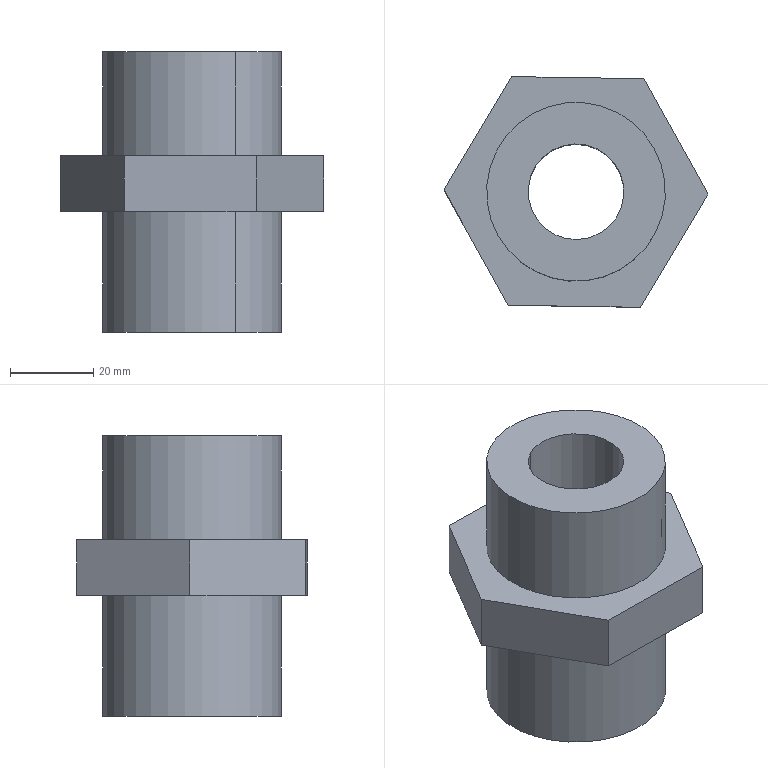Component | SolidWorks | YC1-250-04BalancerAssembly#16673-1_Rc11-4StraightInternalConnection-1 | 1 solid | 16 faces | box 63.5 x 55.49 x 67.5 mm | volume 85682 mm3 | plane 10 | cylinder 6 | commonest cylinder face diameters 43 x4 23 x2 | material Plain Carbon Steel
STEP:
#1=COLOUR_RGB('',0.7922,0.8196,0.9333);
#2=FILL_AREA_STYLE_COLOUR('',#1);
#3=FILL_AREA_STYLE('',(#2));
#4=SURFACE_STYLE_FILL_AREA(#3);
#5=SURFACE_SIDE_STYLE('',(#4));
#6=SURFACE_STYLE_USAGE(.BOTH.,#5);
#7=PRESENTATION_STYLE_ASSIGNMENT((#6));
#8=CARTESIAN_POINT('',(-18.331,156.793,-8.484));
#9=VERTEX_POINT('',#8);
#10=CARTESIAN_POINT('',(-17.89,156.002,-8.484));
#11=VERTEX_POINT('',#10);
#12=CARTESIAN_POINT('',(-18.11,156.398,-8.484));
#13=DIRECTION('',(-0.,-0.,-1.));
#14=DIRECTION('',(-0.8737,-0.4865,0.));
#15=AXIS2_PLACEMENT_3D('',#12,#13,#14);
#16=CIRCLE('',#15,0.4528);
#17=EDGE_CURVE('',#9,#11,#16,.T.);
#18=ORIENTED_EDGE('',*,*,#17,.T.);
#19=CARTESIAN_POINT('',(-17.89,156.002,-5.827));
#20=VERTEX_POINT('',#19);
#21=CARTESIAN_POINT('',(-17.89,156.002,-8.583));
#22=DIRECTION('',(0.,0.,1.));
#23=VECTOR('',#22,39.37);
#24=LINE('',#21,#23);
#25=EDGE_CURVE('',#11,#20,#24,.T.);
#26=ORIENTED_EDGE('',*,*,#25,.T.);
#27=CARTESIAN_POINT('',(-18.331,156.793,-5.827));
#28=VERTEX_POINT('',#27);
#29=CARTESIAN_POINT('',(-18.11,156.398,-5.827));
#30=DIRECTION('',(-0.,-0.,-1.));
#31=DIRECTION('',(-0.4865,0.8737,0.));
#32=AXIS2_PLACEMENT_3D('',#29,#30,#31);
#33=CIRCLE('',#32,0.4528);
#34=EDGE_CURVE('',#28,#20,#33,.T.);
#35=ORIENTED_EDGE('',*,*,#34,.F.);
#36=CARTESIAN_POINT('',(-18.331,156.793,-8.583));
#37=DIRECTION('',(0.,0.,1.));
#38=VECTOR('',#37,39.37);
#39=LINE('',#36,#38);
#40=EDGE_CURVE('',#9,#28,#39,.T.);
#41=ORIENTED_EDGE('',*,*,#40,.F.);
#42=EDGE_LOOP('',(#18,#26,#35,#41));
#43=FACE_OUTER_BOUND('',#42,.T.);
#44=CARTESIAN_POINT('',(-18.11,156.398,-8.583));
#45=DIRECTION('',(0.,0.,1.));
#46=DIRECTION('',(-0.4865,0.8737,0.));
#47=AXIS2_PLACEMENT_3D('',#44,#45,#46);
#48=CYLINDRICAL_SURFACE('',#47,0.4528);
#49=ADVANCED_FACE('',(#43),#48,.F.);
#50=CARTESIAN_POINT('',(-17.698,155.658,-8.484));
#51=VERTEX_POINT('',#50);
#52=CARTESIAN_POINT('',(-18.522,157.137,-8.484));
#53=VERTEX_POINT('',#52);
#54=CARTESIAN_POINT('',(-18.11,156.398,-8.484));
#55=DIRECTION('',(-0.,-0.,-1.));
#56=DIRECTION('',(-0.8737,-0.4865,0.));
#57=AXIS2_PLACEMENT_3D('',#54,#55,#56);
#58=CIRCLE('',#57,0.8465);
#59=EDGE_CURVE('',#51,#53,#58,.T.);
#60=ORIENTED_EDGE('',*,*,#59,.F.);
#61=CARTESIAN_POINT('',(-17.698,155.658,-7.341));
#62=VERTEX_POINT('',#61);
#63=CARTESIAN_POINT('',(-17.698,155.658,-8.583));
#64=DIRECTION('',(0.,0.,1.));
#65=VECTOR('',#64,39.37);
#66=LINE('',#63,#65);
#67=EDGE_CURVE('',#51,#62,#66,.T.);
#68=ORIENTED_EDGE('',*,*,#67,.T.);
#69=CARTESIAN_POINT('',(-18.522,157.137,-7.341));
#70=VERTEX_POINT('',#69);
#71=CARTESIAN_POINT('',(-18.11,156.398,-7.341));
#72=DIRECTION('',(-0.,-0.,-1.));
#73=DIRECTION('',(0.8737,0.4865,0.));
#74=AXIS2_PLACEMENT_3D('',#71,#72,#73);
#75=CIRCLE('',#74,0.8465);
#76=EDGE_CURVE('',#62,#70,#75,.T.);
#77=ORIENTED_EDGE('',*,*,#76,.T.);
#78=CARTESIAN_POINT('',(-18.522,157.137,-8.583));
#79=DIRECTION('',(0.,0.,1.));
#80=VECTOR('',#79,39.37);
#81=LINE('',#78,#80);
#82=EDGE_CURVE('',#53,#70,#81,.T.);
#83=ORIENTED_EDGE('',*,*,#82,.F.);
#84=EDGE_LOOP('',(#60,#68,#77,#83));
#85=FACE_OUTER_BOUND('',#84,.T.);
#86=CARTESIAN_POINT('',(-18.11,156.398,-8.583));
#87=DIRECTION('',(0.,0.,1.));
#88=DIRECTION('',(-0.4865,0.8737,0.));
#89=AXIS2_PLACEMENT_3D('',#86,#87,#88);
#90=CYLINDRICAL_SURFACE('',#89,0.8465);
#91=ADVANCED_FACE('',(#85),#90,.T.);
#92=CARTESIAN_POINT('',(-18.522,157.137,-5.827));
#93=VERTEX_POINT('',#92);
#94=CARTESIAN_POINT('',(-17.698,155.658,-5.827));
#95=VERTEX_POINT('',#94);
#96=CARTESIAN_POINT('',(-18.11,156.398,-5.827));
#97=DIRECTION('',(0.,0.,1.));
#98=DIRECTION('',(0.4865,-0.8737,0.));
#99=AXIS2_PLACEMENT_3D('',#96,#97,#98);
#100=CIRCLE('',#99,0.8465);
#101=EDGE_CURVE('',#93,#95,#100,.T.);
#102=ORIENTED_EDGE('',*,*,#101,.F.);
#103=CARTESIAN_POINT('',(-18.522,157.137,-6.811));
#104=VERTEX_POINT('',#103);
#105=CARTESIAN_POINT('',(-18.522,157.137,-5.827));
#106=DIRECTION('',(-0.,-0.,-1.));
#107=VECTOR('',#106,39.37);
#108=LINE('',#105,#107);
#109=EDGE_CURVE('',#93,#104,#108,.T.);
#110=ORIENTED_EDGE('',*,*,#109,.T.);
#111=CARTESIAN_POINT('',(-17.698,155.658,-6.811));
#112=VERTEX_POINT('',#111);
#113=CARTESIAN_POINT('',(-18.11,156.398,-6.811));
#114=DIRECTION('',(0.,0.,1.));
#115=DIRECTION('',(0.4865,-0.8737,0.));
#116=AXIS2_PLACEMENT_3D('',#113,#114,#115);
#117=CIRCLE('',#116,0.8465);
#118=EDGE_CURVE('',#104,#112,#117,.T.);
#119=ORIENTED_EDGE('',*,*,#118,.T.);
#120=CARTESIAN_POINT('',(-17.698,155.658,-5.827));
#121=DIRECTION('',(-0.,-0.,-1.));
#122=VECTOR('',#121,39.37);
#123=LINE('',#120,#122);
#124=EDGE_CURVE('',#95,#112,#123,.T.);
#125=ORIENTED_EDGE('',*,*,#124,.F.);
#126=EDGE_LOOP('',(#102,#110,#119,#125));
#127=FACE_OUTER_BOUND('',#126,.T.);
#128=CARTESIAN_POINT('',(-18.11,156.398,-5.827));
#129=DIRECTION('',(-0.,-0.,-1.));
#130=DIRECTION('',(0.4865,-0.8737,0.));
#131=AXIS2_PLACEMENT_3D('',#128,#129,#130);
#132=CYLINDRICAL_SURFACE('',#131,0.8465);
#133=ADVANCED_FACE('',(#127),#132,.T.);
#134=ORIENTED_EDGE('',*,*,#25,.F.);
#135=CARTESIAN_POINT('',(-18.11,156.398,-8.484));
#136=DIRECTION('',(-0.,-0.,-1.));
#137=DIRECTION('',(-0.8737,-0.4865,0.));
#138=AXIS2_PLACEMENT_3D('',#135,#136,#137);
#139=CIRCLE('',#138,0.4528);
#140=EDGE_CURVE('',#11,#9,#139,.T.);
#141=ORIENTED_EDGE('',*,*,#140,.T.);
#142=ORIENTED_EDGE('',*,*,#40,.T.);
#143=CARTESIAN_POINT('',(-18.11,156.398,-5.827));
#144=DIRECTION('',(-0.,-0.,-1.));
#145=DIRECTION('',(-0.4865,0.8737,0.));
#146=AXIS2_PLACEMENT_3D('',#143,#144,#145);
#147=CIRCLE('',#146,0.4528);
#148=EDGE_CURVE('',#20,#28,#147,.T.);
#149=ORIENTED_EDGE('',*,*,#148,.F.);
#150=EDGE_LOOP('',(#134,#141,#142,#149));
#151=FACE_OUTER_BOUND('',#150,.T.);
#152=CARTESIAN_POINT('',(-18.11,156.398,-8.583));
#153=DIRECTION('',(0.,0.,1.));
#154=DIRECTION('',(-0.4865,0.8737,0.));
#155=AXIS2_PLACEMENT_3D('',#152,#153,#154);
#156=CYLINDRICAL_SURFACE('',#155,0.4528);
#157=ADVANCED_FACE('',(#151),#156,.F.);
#158=CARTESIAN_POINT('',(-18.11,156.398,-5.827));
#159=DIRECTION('',(0.,0.,1.));
#160=DIRECTION('',(0.4865,-0.8737,0.));
#161=AXIS2_PLACEMENT_3D('',#158,#159,#160);
#162=CIRCLE('',#161,0.8465);
#163=EDGE_CURVE('',#95,#93,#162,.T.);
#164=ORIENTED_EDGE('',*,*,#163,.T.);
#165=ORIENTED_EDGE('',*,*,#101,.T.);
#166=EDGE_LOOP('',(#164,#165));
#167=FACE_OUTER_BOUND('',#166,.T.);
#168=ORIENTED_EDGE('',*,*,#34,.T.);
#169=ORIENTED_EDGE('',*,*,#148,.T.);
#170=EDGE_LOOP('',(#168,#169));
#171=FACE_BOUND('',#170,.T.);
#172=CARTESIAN_POINT('',(-18.11,156.398,-5.827));
#173=DIRECTION('',(0.,0.,1.));
#174=DIRECTION('',(-0.4865,0.8737,-0.));
#175=AXIS2_PLACEMENT_3D('',#172,#173,#174);
#176=PLANE('',#175);
#177=ADVANCED_FACE('',(#167,#171),#176,.T.);
#178=ORIENTED_EDGE('',*,*,#67,.F.);
#179=CARTESIAN_POINT('',(-18.11,156.398,-8.484));
#180=DIRECTION('',(-0.,-0.,-1.));
#181=DIRECTION('',(-0.8737,-0.4865,0.));
#182=AXIS2_PLACEMENT_3D('',#179,#180,#181);
#183=CIRCLE('',#182,0.8465);
#184=EDGE_CURVE('',#53,#51,#183,.T.);
#185=ORIENTED_EDGE('',*,*,#184,.F.);
#186=ORIENTED_EDGE('',*,*,#82,.T.);
#187=CARTESIAN_POINT('',(-18.11,156.398,-7.341));
#188=DIRECTION('',(-0.,-0.,-1.));
#189=DIRECTION('',(0.8737,0.4865,0.));
#190=AXIS2_PLACEMENT_3D('',#187,#188,#189);
#191=CIRCLE('',#190,0.8465);
#192=EDGE_CURVE('',#70,#62,#191,.T.);
#193=ORIENTED_EDGE('',*,*,#192,.T.);
#194=EDGE_LOOP('',(#178,#185,#186,#193));
#195=FACE_OUTER_BOUND('',#194,.T.);
#196=CARTESIAN_POINT('',(-18.11,156.398,-8.583));
#197=DIRECTION('',(0.,0.,1.));
#198=DIRECTION('',(-0.4865,0.8737,0.));
#199=AXIS2_PLACEMENT_3D('',#196,#197,#198);
#200=CYLINDRICAL_SURFACE('',#199,0.8465);
#201=ADVANCED_FACE('',(#195),#200,.T.);
#202=ORIENTED_EDGE('',*,*,#109,.F.);
#203=ORIENTED_EDGE('',*,*,#163,.F.);
#204=ORIENTED_EDGE('',*,*,#124,.T.);
#205=CARTESIAN_POINT('',(-18.11,156.398,-6.811));
#206=DIRECTION('',(0.,0.,1.));
#207=DIRECTION('',(0.4865,-0.8737,0.));
#208=AXIS2_PLACEMENT_3D('',#205,#206,#207);
#209=CIRCLE('',#208,0.8465);
#210=EDGE_CURVE('',#112,#104,#209,.T.);
#211=ORIENTED_EDGE('',*,*,#210,.T.);
#212=EDGE_LOOP('',(#202,#203,#204,#211));
#213=FACE_OUTER_BOUND('',#212,.T.);
#214=CARTESIAN_POINT('',(-18.11,156.398,-5.827));
#215=DIRECTION('',(-0.,-0.,-1.));
#216=DIRECTION('',(0.4865,-0.8737,0.));
#217=AXIS2_PLACEMENT_3D('',#214,#215,#216);
#218=CYLINDRICAL_SURFACE('',#217,0.8465);
#219=ADVANCED_FACE('',(#213),#218,.T.);
#220=ORIENTED_EDGE('',*,*,#210,.F.);
#221=ORIENTED_EDGE('',*,*,#118,.F.);
#222=EDGE_LOOP('',(#220,#221));
#223=FACE_BOUND('',#222,.T.);
#224=CARTESIAN_POINT('',(-19.36,156.417,-6.811));
#225=VERTEX_POINT('',#224);
#226=CARTESIAN_POINT('',(-18.752,155.325,-6.811));
#227=VERTEX_POINT('',#226);
#228=CARTESIAN_POINT('',(-18.752,155.325,-6.811));
#229=DIRECTION('',(0.4865,-0.8737,0.));
#230=VECTOR('',#229,39.37);
#231=LINE('',#228,#230);
#232=EDGE_CURVE('',#225,#227,#231,.T.);
#233=ORIENTED_EDGE('',*,*,#232,.T.);
#234=CARTESIAN_POINT('',(-17.502,155.305,-6.811));
#235=VERTEX_POINT('',#234);
#236=CARTESIAN_POINT('',(-18.752,155.325,-6.811));
#237=DIRECTION('',(0.9999,-0.01552,0.));
#238=VECTOR('',#237,39.37);
#239=LINE('',#236,#238);
#240=EDGE_CURVE('',#227,#235,#239,.T.);
#241=ORIENTED_EDGE('',*,*,#240,.T.);
#242=CARTESIAN_POINT('',(-16.86,156.378,-6.811));
#243=VERTEX_POINT('',#242);
#244=CARTESIAN_POINT('',(-17.502,155.305,-6.811));
#245=DIRECTION('',(0.5134,0.8582,-0.));
#246=VECTOR('',#245,39.37);
#247=LINE('',#244,#246);
#248=EDGE_CURVE('',#235,#243,#247,.T.);
#249=ORIENTED_EDGE('',*,*,#248,.T.);
#250=CARTESIAN_POINT('',(-17.468,157.47,-6.811));
#251=VERTEX_POINT('',#250);
#252=CARTESIAN_POINT('',(-16.86,156.378,-6.811));
#253=DIRECTION('',(-0.4865,0.8737,-0.));
#254=VECTOR('',#253,39.37);
#255=LINE('',#252,#254);
#256=EDGE_CURVE('',#243,#251,#255,.T.);
#257=ORIENTED_EDGE('',*,*,#256,.T.);
#258=CARTESIAN_POINT('',(-18.718,157.49,-6.811));
#259=VERTEX_POINT('',#258);
#260=CARTESIAN_POINT('',(-17.468,157.47,-6.811));
#261=DIRECTION('',(-0.9999,0.01552,-0.));
#262=VECTOR('',#261,39.37);
#263=LINE('',#260,#262);
#264=EDGE_CURVE('',#251,#259,#263,.T.);
#265=ORIENTED_EDGE('',*,*,#264,.T.);
#266=CARTESIAN_POINT('',(-18.718,157.49,-6.811));
#267=DIRECTION('',(-0.5134,-0.8582,0.));
#268=VECTOR('',#267,39.37);
#269=LINE('',#266,#268);
#270=EDGE_CURVE('',#259,#225,#269,.T.);
#271=ORIENTED_EDGE('',*,*,#270,.T.);
#272=EDGE_LOOP('',(#233,#241,#249,#257,#265,#271));
#273=FACE_OUTER_BOUND('',#272,.T.);
#274=CARTESIAN_POINT('',(-16.86,156.378,-6.811));
#275=DIRECTION('',(0.,0.,1.));
#276=DIRECTION('',(-0.4865,0.8737,-0.));
#277=AXIS2_PLACEMENT_3D('',#274,#275,#276);
#278=PLANE('',#277);
#279=ADVANCED_FACE('',(#223,#273),#278,.T.);
#280=CARTESIAN_POINT('',(-17.502,155.305,-7.341));
#281=VERTEX_POINT('',#280);
#282=CARTESIAN_POINT('',(-17.502,155.305,-6.811));
#283=DIRECTION('',(0.,0.,1.));
#284=VECTOR('',#283,39.37);
#285=LINE('',#282,#284);
#286=EDGE_CURVE('',#281,#235,#285,.T.);
#287=ORIENTED_EDGE('',*,*,#286,.F.);
#288=CARTESIAN_POINT('',(-16.86,156.378,-7.341));
#289=VERTEX_POINT('',#288);
#290=CARTESIAN_POINT('',(-17.502,155.305,-7.341));
#291=DIRECTION('',(0.5134,0.8582,-0.));
#292=VECTOR('',#291,39.37);
#293=LINE('',#290,#292);
#294=EDGE_CURVE('',#281,#289,#293,.T.);
#295=ORIENTED_EDGE('',*,*,#294,.T.);
#296=CARTESIAN_POINT('',(-16.86,156.378,-6.811));
#297=DIRECTION('',(-0.,-0.,-1.));
#298=VECTOR('',#297,39.37);
#299=LINE('',#296,#298);
#300=EDGE_CURVE('',#243,#289,#299,.T.);
#301=ORIENTED_EDGE('',*,*,#300,.F.);
#302=ORIENTED_EDGE('',*,*,#248,.F.);
#303=EDGE_LOOP('',(#287,#295,#301,#302));
#304=FACE_OUTER_BOUND('',#303,.T.);
#305=CARTESIAN_POINT('',(-17.502,155.305,-6.811));
#306=DIRECTION('',(-0.8582,0.5134,-0.));
#307=DIRECTION('',(-0.5134,-0.8582,0.));
#308=AXIS2_PLACEMENT_3D('',#305,#306,#307);
#309=PLANE('',#308);
#310=ADVANCED_FACE('',(#304),#309,.F.);
#311=CARTESIAN_POINT('',(-18.752,155.325,-7.341));
#312=VERTEX_POINT('',#311);
#313=CARTESIAN_POINT('',(-18.752,155.325,-6.811));
#314=DIRECTION('',(0.,0.,1.));
#315=VECTOR('',#314,39.37);
#316=LINE('',#313,#315);
#317=EDGE_CURVE('',#312,#227,#316,.T.);
#318=ORIENTED_EDGE('',*,*,#317,.F.);
#319=CARTESIAN_POINT('',(-18.752,155.325,-7.341));
#320=DIRECTION('',(0.9999,-0.01552,0.));
#321=VECTOR('',#320,39.37);
#322=LINE('',#319,#321);
#323=EDGE_CURVE('',#312,#281,#322,.T.);
#324=ORIENTED_EDGE('',*,*,#323,.T.);
#325=ORIENTED_EDGE('',*,*,#286,.T.);
#326=ORIENTED_EDGE('',*,*,#240,.F.);
#327=EDGE_LOOP('',(#318,#324,#325,#326));
#328=FACE_OUTER_BOUND('',#327,.T.);
#329=CARTESIAN_POINT('',(-18.752,155.325,-6.811));
#330=DIRECTION('',(0.01552,0.9999,-0.));
#331=DIRECTION('',(-0.9999,0.01552,-0.));
#332=AXIS2_PLACEMENT_3D('',#329,#330,#331);
#333=PLANE('',#332);
#334=ADVANCED_FACE('',(#328),#333,.F.);
#335=CARTESIAN_POINT('',(-19.36,156.417,-7.341));
#336=VERTEX_POINT('',#335);
#337=CARTESIAN_POINT('',(-19.36,156.417,-6.811));
#338=DIRECTION('',(0.,0.,1.));
#339=VECTOR('',#338,39.37);
#340=LINE('',#337,#339);
#341=EDGE_CURVE('',#336,#225,#340,.T.);
#342=ORIENTED_EDGE('',*,*,#341,.F.);
#343=CARTESIAN_POINT('',(-19.36,156.417,-7.341));
#344=DIRECTION('',(0.4865,-0.8737,0.));
#345=VECTOR('',#344,39.37);
#346=LINE('',#343,#345);
#347=EDGE_CURVE('',#336,#312,#346,.T.);
#348=ORIENTED_EDGE('',*,*,#347,.T.);
#349=ORIENTED_EDGE('',*,*,#317,.T.);
#350=ORIENTED_EDGE('',*,*,#232,.F.);
#351=EDGE_LOOP('',(#342,#348,#349,#350));
#352=FACE_OUTER_BOUND('',#351,.T.);
#353=CARTESIAN_POINT('',(-19.36,156.417,-6.811));
#354=DIRECTION('',(0.8737,0.4865,-0.));
#355=DIRECTION('',(-0.4865,0.8737,-0.));
#356=AXIS2_PLACEMENT_3D('',#353,#354,#355);
#357=PLANE('',#356);
#358=ADVANCED_FACE('',(#352),#357,.F.);
#359=CARTESIAN_POINT('',(-18.718,157.49,-7.341));
#360=VERTEX_POINT('',#359);
#361=CARTESIAN_POINT('',(-18.718,157.49,-6.811));
#362=DIRECTION('',(0.,0.,1.));
#363=VECTOR('',#362,39.37);
#364=LINE('',#361,#363);
#365=EDGE_CURVE('',#360,#259,#364,.T.);
#366=ORIENTED_EDGE('',*,*,#365,.F.);
#367=CARTESIAN_POINT('',(-18.718,157.49,-7.341));
#368=DIRECTION('',(-0.5134,-0.8582,0.));
#369=VECTOR('',#368,39.37);
#370=LINE('',#367,#369);
#371=EDGE_CURVE('',#360,#336,#370,.T.);
#372=ORIENTED_EDGE('',*,*,#371,.T.);
#373=ORIENTED_EDGE('',*,*,#341,.T.);
#374=ORIENTED_EDGE('',*,*,#270,.F.);
#375=EDGE_LOOP('',(#366,#372,#373,#374));
#376=FACE_OUTER_BOUND('',#375,.T.);
#377=CARTESIAN_POINT('',(-18.718,157.49,-6.811));
#378=DIRECTION('',(0.8582,-0.5134,0.));
#379=DIRECTION('',(0.5134,0.8582,-0.));
#380=AXIS2_PLACEMENT_3D('',#377,#378,#379);
#381=PLANE('',#380);
#382=ADVANCED_FACE('',(#376),#381,.F.);
#383=CARTESIAN_POINT('',(-17.468,157.47,-7.341));
#384=VERTEX_POINT('',#383);
#385=CARTESIAN_POINT('',(-17.468,157.47,-6.811));
#386=DIRECTION('',(0.,0.,1.));
#387=VECTOR('',#386,39.37);
#388=LINE('',#385,#387);
#389=EDGE_CURVE('',#384,#251,#388,.T.);
#390=ORIENTED_EDGE('',*,*,#389,.F.);
#391=CARTESIAN_POINT('',(-17.468,157.47,-7.341));
#392=DIRECTION('',(-0.9999,0.01552,-0.));
#393=VECTOR('',#392,39.37);
#394=LINE('',#391,#393);
#395=EDGE_CURVE('',#384,#360,#394,.T.);
#396=ORIENTED_EDGE('',*,*,#395,.T.);
#397=ORIENTED_EDGE('',*,*,#365,.T.);
#398=ORIENTED_EDGE('',*,*,#264,.F.);
#399=EDGE_LOOP('',(#390,#396,#397,#398));
#400=FACE_OUTER_BOUND('',#399,.T.);
#401=CARTESIAN_POINT('',(-17.468,157.47,-6.811));
#402=DIRECTION('',(-0.01552,-0.9999,0.));
#403=DIRECTION('',(0.9999,-0.01552,0.));
#404=AXIS2_PLACEMENT_3D('',#401,#402,#403);
#405=PLANE('',#404);
#406=ADVANCED_FACE('',(#400),#405,.F.);
#407=ORIENTED_EDGE('',*,*,#300,.T.);
#408=CARTESIAN_POINT('',(-16.86,156.378,-7.341));
#409=DIRECTION('',(-0.4865,0.8737,-0.));
#410=VECTOR('',#409,39.37);
#411=LINE('',#408,#410);
#412=EDGE_CURVE('',#289,#384,#411,.T.);
#413=ORIENTED_EDGE('',*,*,#412,.T.);
#414=ORIENTED_EDGE('',*,*,#389,.T.);
#415=ORIENTED_EDGE('',*,*,#256,.F.);
#416=EDGE_LOOP('',(#407,#413,#414,#415));
#417=FACE_OUTER_BOUND('',#416,.T.);
#418=CARTESIAN_POINT('',(-16.86,156.378,-6.811));
#419=DIRECTION('',(-0.8737,-0.4865,0.));
#420=DIRECTION('',(0.4865,-0.8737,0.));
#421=AXIS2_PLACEMENT_3D('',#418,#419,#420);
#422=PLANE('',#421);
#423=ADVANCED_FACE('',(#417),#422,.F.);
#424=ORIENTED_EDGE('',*,*,#192,.F.);
#425=ORIENTED_EDGE('',*,*,#76,.F.);
#426=EDGE_LOOP('',(#424,#425));
#427=FACE_BOUND('',#426,.T.);
#428=ORIENTED_EDGE('',*,*,#294,.F.);
#429=ORIENTED_EDGE('',*,*,#323,.F.);
#430=ORIENTED_EDGE('',*,*,#347,.F.);
#431=ORIENTED_EDGE('',*,*,#371,.F.);
#432=ORIENTED_EDGE('',*,*,#395,.F.);
#433=ORIENTED_EDGE('',*,*,#412,.F.);
#434=EDGE_LOOP('',(#428,#429,#430,#431,#432,#433));
#435=FACE_OUTER_BOUND('',#434,.T.);
#436=CARTESIAN_POINT('',(-17.344,155.022,-7.341));
#437=DIRECTION('',(0.,0.,1.));
#438=DIRECTION('',(-0.8737,-0.4865,0.));
#439=AXIS2_PLACEMENT_3D('',#436,#437,#438);
#440=PLANE('',#439);
#441=ADVANCED_FACE('',(#427,#435),#440,.F.);
#442=ORIENTED_EDGE('',*,*,#184,.T.);
#443=ORIENTED_EDGE('',*,*,#59,.T.);
#444=EDGE_LOOP('',(#442,#443));
#445=FACE_OUTER_BOUND('',#444,.T.);
#446=ORIENTED_EDGE('',*,*,#17,.F.);
#447=ORIENTED_EDGE('',*,*,#140,.F.);
#448=EDGE_LOOP('',(#446,#447));
#449=FACE_BOUND('',#448,.T.);
#450=CARTESIAN_POINT('',(-17.631,155.538,-8.484));
#451=DIRECTION('',(0.,0.,1.));
#452=DIRECTION('',(-0.8737,-0.4865,0.));
#453=AXIS2_PLACEMENT_3D('',#450,#451,#452);
#454=PLANE('',#453);
#455=ADVANCED_FACE('',(#445,#449),#454,.F.);
#456=CLOSED_SHELL('',(#49,#91,#133,#157,#177,#201,#219,#279,#310,#334,#358,#382,#406,#423,#441,#455));
#457=MANIFOLD_SOLID_BREP('',#456);
#458=STYLED_ITEM('',(#7),#457);
#459=PRESENTATION_LAYER_ASSIGNMENT('','',(#458));
#460=CARTESIAN_POINT('',(0.,0.,0.));
#461=DIRECTION('',(0.,0.,1.));
#462=DIRECTION('',(1.,0.,0.));
#463=AXIS2_PLACEMENT_3D('',#460,#461,#462);
#464=(LENGTH_UNIT()NAMED_UNIT(*)SI_UNIT($,.METRE.));
#465=LENGTH_MEASURE_WITH_UNIT(LENGTH_MEASURE(0.0254),#464);
#466=DIMENSIONAL_EXPONENTS(1.,0.,0.,0.,0.,0.,0.);
#467=(CONVERSION_BASED_UNIT('',#465)LENGTH_UNIT()NAMED_UNIT(#466));
#468=UNCERTAINTY_MEASURE_WITH_UNIT(LENGTH_MEASURE(0.00001),#467,'','');
#469=(NAMED_UNIT(*)PLANE_ANGLE_UNIT()SI_UNIT($,.RADIAN.));
#470=(NAMED_UNIT(*)SI_UNIT($,.STERADIAN.)SOLID_ANGLE_UNIT());
#471=(GEOMETRIC_REPRESENTATION_CONTEXT(3)GLOBAL_UNCERTAINTY_ASSIGNED_CONTEXT((#468))GLOBAL_UNIT_ASSIGNED_CONTEXT((#467,#469,#470))REPRESENTATION_CONTEXT('',''));
#472=ADVANCED_BREP_SHAPE_REPRESENTATION('',(#457,#463),#471);
#473=(LENGTH_UNIT()NAMED_UNIT(*)SI_UNIT($,.METRE.));
#474=LENGTH_MEASURE_WITH_UNIT(LENGTH_MEASURE(0.0254),#473);
#475=DIMENSIONAL_EXPONENTS(1.,0.,0.,0.,0.,0.,0.);
#476=(CONVERSION_BASED_UNIT('',#474)LENGTH_UNIT()NAMED_UNIT(#475));
#477=UNCERTAINTY_MEASURE_WITH_UNIT(LENGTH_MEASURE(0.00001),#476,'','');
#478=(NAMED_UNIT(*)PLANE_ANGLE_UNIT()SI_UNIT($,.RADIAN.));
#479=(NAMED_UNIT(*)SI_UNIT($,.STERADIAN.)SOLID_ANGLE_UNIT());
#480=(GEOMETRIC_REPRESENTATION_CONTEXT(3)GLOBAL_UNCERTAINTY_ASSIGNED_CONTEXT((#477))GLOBAL_UNIT_ASSIGNED_CONTEXT((#476,#478,#479))REPRESENTATION_CONTEXT('',''));
#481=MECHANICAL_DESIGN_GEOMETRIC_PRESENTATION_REPRESENTATION('',(#458),#480);